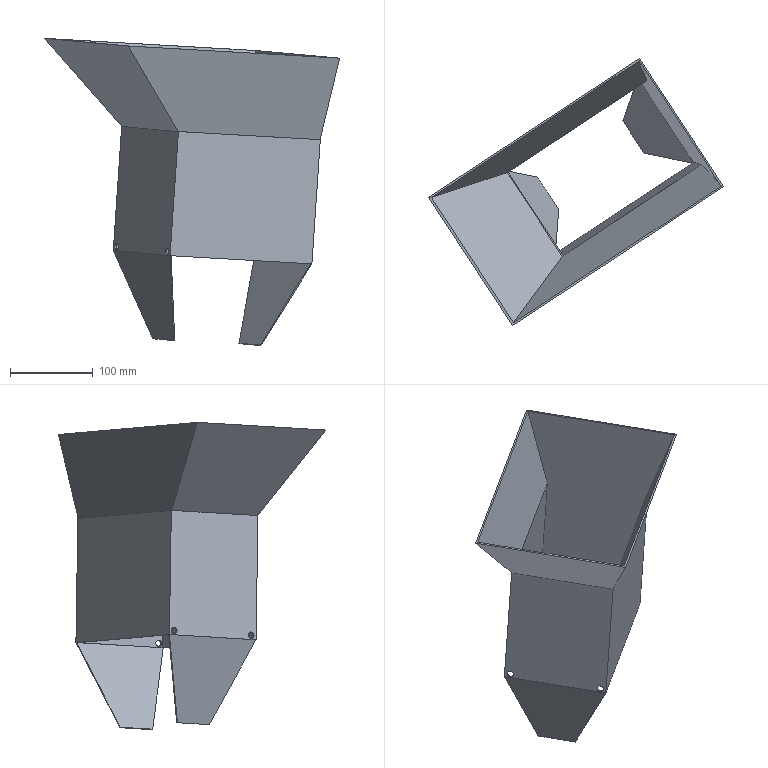Component | SolidWorks | MaterialChannel-1 | 1 solid | 37 faces | box 355.68 x 322.15 x 370.35 mm | volume 401352 mm3 | plane 29 | cylinder 8 | commonest cylinder face diameters 8 x8 | material AISI 304
STEP:
#1=COLOUR_RGB('',0.7922,0.8196,0.9333);
#2=FILL_AREA_STYLE_COLOUR('',#1);
#3=FILL_AREA_STYLE('',(#2));
#4=SURFACE_STYLE_FILL_AREA(#3);
#5=SURFACE_SIDE_STYLE('',(#4));
#6=SURFACE_STYLE_USAGE(.BOTH.,#5);
#7=PRESENTATION_STYLE_ASSIGNMENT((#6));
#8=CARTESIAN_POINT('',(-10.12,-1.207,26.784));
#9=VERTEX_POINT('',#8);
#10=CARTESIAN_POINT('',(-10.292,-0.9443,26.8));
#11=VERTEX_POINT('',#10);
#12=CARTESIAN_POINT('',(-10.206,-1.076,26.792));
#13=DIRECTION('',(0.8341,0.5496,-0.04788));
#14=DIRECTION('',(-0.5475,0.8353,0.05005));
#15=AXIS2_PLACEMENT_3D('',#12,#13,#14);
#16=CIRCLE('',#15,0.1575);
#17=EDGE_CURVE('',#9,#11,#16,.T.);
#18=ORIENTED_EDGE('',*,*,#17,.T.);
#19=CARTESIAN_POINT('',(-10.358,-0.9876,26.804));
#20=VERTEX_POINT('',#19);
#21=CARTESIAN_POINT('',(-3.626,3.448,26.418));
#22=DIRECTION('',(-0.8341,-0.5496,0.04788));
#23=VECTOR('',#22,39.37);
#24=LINE('',#21,#23);
#25=EDGE_CURVE('',#11,#20,#24,.T.);
#26=ORIENTED_EDGE('',*,*,#25,.T.);
#27=CARTESIAN_POINT('',(-10.186,-1.251,26.788));
#28=VERTEX_POINT('',#27);
#29=CARTESIAN_POINT('',(-10.272,-1.119,26.796));
#30=DIRECTION('',(-0.8341,-0.5496,0.04788));
#31=DIRECTION('',(0.5475,-0.8353,-0.05005));
#32=AXIS2_PLACEMENT_3D('',#29,#30,#31);
#33=CIRCLE('',#32,0.1575);
#34=EDGE_CURVE('',#20,#28,#33,.T.);
#35=ORIENTED_EDGE('',*,*,#34,.T.);
#36=CARTESIAN_POINT('',(-3.454,3.185,26.402));
#37=DIRECTION('',(-0.8341,-0.5496,0.04788));
#38=VECTOR('',#37,39.37);
#39=LINE('',#36,#38);
#40=EDGE_CURVE('',#9,#28,#39,.T.);
#41=ORIENTED_EDGE('',*,*,#40,.F.);
#42=EDGE_LOOP('',(#18,#26,#35,#41));
#43=FACE_OUTER_BOUND('',#42,.T.);
#44=CARTESIAN_POINT('',(-3.54,3.317,26.41));
#45=DIRECTION('',(-0.8341,-0.5496,0.04788));
#46=DIRECTION('',(0.5475,-0.8353,-0.05005));
#47=AXIS2_PLACEMENT_3D('',#44,#45,#46);
#48=CYLINDRICAL_SURFACE('',#47,0.1575);
#49=ADVANCED_FACE('',(#43),#48,.F.);
#50=CARTESIAN_POINT('',(-3.626,3.448,26.418));
#51=VERTEX_POINT('',#50);
#52=CARTESIAN_POINT('',(-3.454,3.185,26.402));
#53=VERTEX_POINT('',#52);
#54=CARTESIAN_POINT('',(-3.54,3.317,26.41));
#55=DIRECTION('',(-0.8341,-0.5496,0.04788));
#56=DIRECTION('',(0.5475,-0.8353,-0.05005));
#57=AXIS2_PLACEMENT_3D('',#54,#55,#56);
#58=CIRCLE('',#57,0.1575);
#59=EDGE_CURVE('',#51,#53,#58,.T.);
#60=ORIENTED_EDGE('',*,*,#59,.F.);
#61=CARTESIAN_POINT('',(-3.692,3.405,26.421));
#62=VERTEX_POINT('',#61);
#63=CARTESIAN_POINT('',(-3.626,3.448,26.418));
#64=DIRECTION('',(-0.8341,-0.5496,0.04788));
#65=VECTOR('',#64,39.37);
#66=LINE('',#63,#65);
#67=EDGE_CURVE('',#51,#62,#66,.T.);
#68=ORIENTED_EDGE('',*,*,#67,.T.);
#69=CARTESIAN_POINT('',(-3.52,3.142,26.406));
#70=VERTEX_POINT('',#69);
#71=CARTESIAN_POINT('',(-3.606,3.273,26.413));
#72=DIRECTION('',(-0.8341,-0.5496,0.04788));
#73=DIRECTION('',(0.5475,-0.8353,-0.05005));
#74=AXIS2_PLACEMENT_3D('',#71,#72,#73);
#75=CIRCLE('',#74,0.1575);
#76=EDGE_CURVE('',#62,#70,#75,.T.);
#77=ORIENTED_EDGE('',*,*,#76,.T.);
#78=CARTESIAN_POINT('',(-3.454,3.185,26.402));
#79=DIRECTION('',(-0.8341,-0.5496,0.04788));
#80=VECTOR('',#79,39.37);
#81=LINE('',#78,#80);
#82=EDGE_CURVE('',#53,#70,#81,.T.);
#83=ORIENTED_EDGE('',*,*,#82,.F.);
#84=EDGE_LOOP('',(#60,#68,#77,#83));
#85=FACE_OUTER_BOUND('',#84,.T.);
#86=CARTESIAN_POINT('',(-3.54,3.317,26.41));
#87=DIRECTION('',(-0.8341,-0.5496,0.04788));
#88=DIRECTION('',(0.5475,-0.8353,-0.05005));
#89=AXIS2_PLACEMENT_3D('',#86,#87,#88);
#90=CYLINDRICAL_SURFACE('',#89,0.1575);
#91=ADVANCED_FACE('',(#85),#90,.F.);
#92=CARTESIAN_POINT('',(-12.513,2.443,27.003));
#93=VERTEX_POINT('',#92);
#94=CARTESIAN_POINT('',(-12.685,2.706,27.019));
#95=VERTEX_POINT('',#94);
#96=CARTESIAN_POINT('',(-12.599,2.574,27.011));
#97=DIRECTION('',(0.8341,0.5496,-0.04788));
#98=DIRECTION('',(-0.5475,0.8353,0.05005));
#99=AXIS2_PLACEMENT_3D('',#96,#97,#98);
#100=CIRCLE('',#99,0.1575);
#101=EDGE_CURVE('',#93,#95,#100,.T.);
#102=ORIENTED_EDGE('',*,*,#101,.T.);
#103=CARTESIAN_POINT('',(-12.751,2.663,27.023));
#104=VERTEX_POINT('',#103);
#105=CARTESIAN_POINT('',(-6.019,7.098,26.636));
#106=DIRECTION('',(-0.8341,-0.5496,0.04788));
#107=VECTOR('',#106,39.37);
#108=LINE('',#105,#107);
#109=EDGE_CURVE('',#95,#104,#108,.T.);
#110=ORIENTED_EDGE('',*,*,#109,.T.);
#111=CARTESIAN_POINT('',(-12.578,2.4,27.007));
#112=VERTEX_POINT('',#111);
#113=CARTESIAN_POINT('',(-12.664,2.531,27.015));
#114=DIRECTION('',(-0.8341,-0.5496,0.04788));
#115=DIRECTION('',(0.5475,-0.8353,-0.05005));
#116=AXIS2_PLACEMENT_3D('',#113,#114,#115);
#117=CIRCLE('',#116,0.1575);
#118=EDGE_CURVE('',#104,#112,#117,.T.);
#119=ORIENTED_EDGE('',*,*,#118,.T.);
#120=CARTESIAN_POINT('',(-5.847,6.835,26.621));
#121=DIRECTION('',(-0.8341,-0.5496,0.04788));
#122=VECTOR('',#121,39.37);
#123=LINE('',#120,#122);
#124=EDGE_CURVE('',#93,#112,#123,.T.);
#125=ORIENTED_EDGE('',*,*,#124,.F.);
#126=EDGE_LOOP('',(#102,#110,#119,#125));
#127=FACE_OUTER_BOUND('',#126,.T.);
#128=CARTESIAN_POINT('',(-5.933,6.967,26.628));
#129=DIRECTION('',(-0.8341,-0.5496,0.04788));
#130=DIRECTION('',(0.5475,-0.8353,-0.05005));
#131=AXIS2_PLACEMENT_3D('',#128,#129,#130);
#132=CYLINDRICAL_SURFACE('',#131,0.1575);
#133=ADVANCED_FACE('',(#127),#132,.F.);
#134=CARTESIAN_POINT('',(-6.019,7.098,26.636));
#135=VERTEX_POINT('',#134);
#136=CARTESIAN_POINT('',(-5.847,6.835,26.621));
#137=VERTEX_POINT('',#136);
#138=CARTESIAN_POINT('',(-5.933,6.967,26.628));
#139=DIRECTION('',(-0.8341,-0.5496,0.04788));
#140=DIRECTION('',(0.5475,-0.8353,-0.05005));
#141=AXIS2_PLACEMENT_3D('',#138,#139,#140);
#142=CIRCLE('',#141,0.1575);
#143=EDGE_CURVE('',#135,#137,#142,.T.);
#144=ORIENTED_EDGE('',*,*,#143,.F.);
#145=CARTESIAN_POINT('',(-6.085,7.055,26.64));
#146=VERTEX_POINT('',#145);
#147=CARTESIAN_POINT('',(-6.019,7.098,26.636));
#148=DIRECTION('',(-0.8341,-0.5496,0.04788));
#149=VECTOR('',#148,39.37);
#150=LINE('',#147,#149);
#151=EDGE_CURVE('',#135,#146,#150,.T.);
#152=ORIENTED_EDGE('',*,*,#151,.T.);
#153=CARTESIAN_POINT('',(-5.912,6.792,26.624));
#154=VERTEX_POINT('',#153);
#155=CARTESIAN_POINT('',(-5.999,6.924,26.632));
#156=DIRECTION('',(-0.8341,-0.5496,0.04788));
#157=DIRECTION('',(0.5475,-0.8353,-0.05005));
#158=AXIS2_PLACEMENT_3D('',#155,#156,#157);
#159=CIRCLE('',#158,0.1575);
#160=EDGE_CURVE('',#146,#154,#159,.T.);
#161=ORIENTED_EDGE('',*,*,#160,.T.);
#162=CARTESIAN_POINT('',(-5.847,6.835,26.621));
#163=DIRECTION('',(-0.8341,-0.5496,0.04788));
#164=VECTOR('',#163,39.37);
#165=LINE('',#162,#164);
#166=EDGE_CURVE('',#137,#154,#165,.T.);
#167=ORIENTED_EDGE('',*,*,#166,.F.);
#168=EDGE_LOOP('',(#144,#152,#161,#167));
#169=FACE_OUTER_BOUND('',#168,.T.);
#170=CARTESIAN_POINT('',(-5.933,6.967,26.628));
#171=DIRECTION('',(-0.8341,-0.5496,0.04788));
#172=DIRECTION('',(0.5475,-0.8353,-0.05005));
#173=AXIS2_PLACEMENT_3D('',#170,#171,#172);
#174=CYLINDRICAL_SURFACE('',#173,0.1575);
#175=ADVANCED_FACE('',(#169),#174,.F.);
#176=CARTESIAN_POINT('',(-9.708,-1.33,32.556));
#177=VERTEX_POINT('',#176);
#178=CARTESIAN_POINT('',(-3.107,3.019,32.177));
#179=VERTEX_POINT('',#178);
#180=CARTESIAN_POINT('',(-3.107,3.019,32.177));
#181=DIRECTION('',(0.8341,0.5496,-0.04788));
#182=VECTOR('',#181,39.37);
#183=LINE('',#180,#182);
#184=EDGE_CURVE('',#177,#179,#183,.T.);
#185=ORIENTED_EDGE('',*,*,#184,.F.);
#186=CARTESIAN_POINT('',(-12.316,2.649,32.794));
#187=VERTEX_POINT('',#186);
#188=CARTESIAN_POINT('',(-9.708,-1.33,32.556));
#189=DIRECTION('',(0.5475,-0.8353,-0.05005));
#190=VECTOR('',#189,39.37);
#191=LINE('',#188,#190);
#192=EDGE_CURVE('',#187,#177,#191,.T.);
#193=ORIENTED_EDGE('',*,*,#192,.F.);
#194=CARTESIAN_POINT('',(-5.716,6.998,32.416));
#195=VERTEX_POINT('',#194);
#196=CARTESIAN_POINT('',(-12.316,2.649,32.794));
#197=DIRECTION('',(-0.8341,-0.5496,0.04788));
#198=VECTOR('',#197,39.37);
#199=LINE('',#196,#198);
#200=EDGE_CURVE('',#195,#187,#199,.T.);
#201=ORIENTED_EDGE('',*,*,#200,.F.);
#202=CARTESIAN_POINT('',(-5.716,6.999,32.416));
#203=VERTEX_POINT('',#202);
#204=CARTESIAN_POINT('',(-5.759,7.064,32.419));
#205=DIRECTION('',(0.5475,-0.8353,-0.05005));
#206=VECTOR('',#205,39.37);
#207=LINE('',#204,#206);
#208=EDGE_CURVE('',#203,#195,#207,.T.);
#209=ORIENTED_EDGE('',*,*,#208,.F.);
#210=CARTESIAN_POINT('',(-12.355,2.624,32.797));
#211=VERTEX_POINT('',#210);
#212=CARTESIAN_POINT('',(-15.666,0.4426,32.987));
#213=DIRECTION('',(0.8341,0.5496,-0.04788));
#214=VECTOR('',#213,39.37);
#215=LINE('',#212,#214);
#216=EDGE_CURVE('',#211,#203,#215,.T.);
#217=ORIENTED_EDGE('',*,*,#216,.F.);
#218=CARTESIAN_POINT('',(-9.746,-1.356,32.558));
#219=VERTEX_POINT('',#218);
#220=CARTESIAN_POINT('',(-9.714,-1.405,32.555));
#221=DIRECTION('',(0.5475,-0.8353,-0.05005));
#222=VECTOR('',#221,39.37);
#223=LINE('',#220,#222);
#224=EDGE_CURVE('',#211,#219,#223,.T.);
#225=ORIENTED_EDGE('',*,*,#224,.T.);
#226=CARTESIAN_POINT('',(-3.107,3.018,32.177));
#227=VERTEX_POINT('',#226);
#228=CARTESIAN_POINT('',(-13.057,-3.538,32.748));
#229=DIRECTION('',(-0.8341,-0.5496,0.04788));
#230=VECTOR('',#229,39.37);
#231=LINE('',#228,#230);
#232=EDGE_CURVE('',#227,#219,#231,.T.);
#233=ORIENTED_EDGE('',*,*,#232,.F.);
#234=CARTESIAN_POINT('',(-5.759,7.064,32.419));
#235=DIRECTION('',(0.5475,-0.8353,-0.05005));
#236=VECTOR('',#235,39.37);
#237=LINE('',#234,#236);
#238=EDGE_CURVE('',#179,#227,#237,.T.);
#239=ORIENTED_EDGE('',*,*,#238,.F.);
#240=EDGE_LOOP('',(#185,#193,#201,#209,#217,#225,#233,#239));
#241=FACE_OUTER_BOUND('',#240,.T.);
#242=CARTESIAN_POINT('',(-13.025,-3.586,32.745));
#243=DIRECTION('',(-0.0675,0.01553,-0.9976));
#244=DIRECTION('',(-0.8341,-0.5496,0.04788));
#245=AXIS2_PLACEMENT_3D('',#242,#243,#244);
#246=PLANE('',#245);
#247=ADVANCED_FACE('',(#241),#246,.F.);
#248=CARTESIAN_POINT('',(-6.079,8.034,36.324));
#249=VERTEX_POINT('',#248);
#250=CARTESIAN_POINT('',(-2.091,1.95,35.959));
#251=VERTEX_POINT('',#250);
#252=CARTESIAN_POINT('',(-2.091,1.95,35.959));
#253=DIRECTION('',(0.5475,-0.8353,-0.05005));
#254=VECTOR('',#253,39.37);
#255=LINE('',#252,#254);
#256=EDGE_CURVE('',#249,#251,#255,.T.);
#257=ORIENTED_EDGE('',*,*,#256,.F.);
#258=CARTESIAN_POINT('',(-16.095,1.434,36.899));
#259=VERTEX_POINT('',#258);
#260=CARTESIAN_POINT('',(-16.095,1.434,36.899));
#261=DIRECTION('',(0.8341,0.5496,-0.04788));
#262=VECTOR('',#261,39.37);
#263=LINE('',#260,#262);
#264=EDGE_CURVE('',#259,#249,#263,.T.);
#265=ORIENTED_EDGE('',*,*,#264,.F.);
#266=CARTESIAN_POINT('',(-12.107,-4.649,36.534));
#267=VERTEX_POINT('',#266);
#268=CARTESIAN_POINT('',(-12.107,-4.649,36.534));
#269=DIRECTION('',(0.5475,-0.8353,-0.05005));
#270=VECTOR('',#269,39.37);
#271=LINE('',#268,#270);
#272=EDGE_CURVE('',#259,#267,#271,.T.);
#273=ORIENTED_EDGE('',*,*,#272,.T.);
#274=CARTESIAN_POINT('',(-12.107,-4.649,36.534));
#275=DIRECTION('',(0.8341,0.5496,-0.04788));
#276=VECTOR('',#275,39.37);
#277=LINE('',#274,#276);
#278=EDGE_CURVE('',#267,#251,#277,.T.);
#279=ORIENTED_EDGE('',*,*,#278,.T.);
#280=EDGE_LOOP('',(#257,#265,#273,#279));
#281=FACE_OUTER_BOUND('',#280,.T.);
#282=CARTESIAN_POINT('',(-15.957,1.427,36.889));
#283=VERTEX_POINT('',#282);
#284=CARTESIAN_POINT('',(-6.1,7.922,36.323));
#285=VERTEX_POINT('',#284);
#286=CARTESIAN_POINT('',(-16.05,1.366,36.895));
#287=DIRECTION('',(0.8341,0.5496,-0.04788));
#288=VECTOR('',#287,39.37);
#289=LINE('',#286,#288);
#290=EDGE_CURVE('',#283,#285,#289,.T.);
#291=ORIENTED_EDGE('',*,*,#290,.T.);
#292=CARTESIAN_POINT('',(-2.202,1.975,35.967));
#293=VERTEX_POINT('',#292);
#294=CARTESIAN_POINT('',(-2.157,1.907,35.963));
#295=DIRECTION('',(0.5475,-0.8353,-0.05005));
#296=VECTOR('',#295,39.37);
#297=LINE('',#294,#296);
#298=EDGE_CURVE('',#285,#293,#297,.T.);
#299=ORIENTED_EDGE('',*,*,#298,.T.);
#300=CARTESIAN_POINT('',(-12.059,-4.519,36.533));
#301=VERTEX_POINT('',#300);
#302=CARTESIAN_POINT('',(-12.152,-4.581,36.538));
#303=DIRECTION('',(0.8341,0.5496,-0.04788));
#304=VECTOR('',#303,39.37);
#305=LINE('',#302,#304);
#306=EDGE_CURVE('',#301,#293,#305,.T.);
#307=ORIENTED_EDGE('',*,*,#306,.F.);
#308=CARTESIAN_POINT('',(-11.691,-5.081,36.499));
#309=DIRECTION('',(0.5475,-0.8353,-0.05005));
#310=VECTOR('',#309,39.37);
#311=LINE('',#308,#310);
#312=EDGE_CURVE('',#283,#301,#311,.T.);
#313=ORIENTED_EDGE('',*,*,#312,.F.);
#314=EDGE_LOOP('',(#291,#299,#307,#313));
#315=FACE_BOUND('',#314,.T.);
#316=CARTESIAN_POINT('',(-12.107,-4.649,36.534));
#317=DIRECTION('',(0.0675,-0.01553,0.9976));
#318=DIRECTION('',(0.8341,0.5496,-0.04788));
#319=AXIS2_PLACEMENT_3D('',#316,#317,#318);
#320=PLANE('',#319);
#321=ADVANCED_FACE('',(#281,#315),#320,.T.);
#322=CARTESIAN_POINT('',(-12.43,2.673,32.724));
#323=VERTEX_POINT('',#322);
#324=CARTESIAN_POINT('',(-12.419,2.656,32.723));
#325=VERTEX_POINT('',#324);
#326=CARTESIAN_POINT('',(-12.43,2.673,32.724));
#327=DIRECTION('',(0.5475,-0.8353,-0.05005));
#328=VECTOR('',#327,39.37);
#329=LINE('',#326,#328);
#330=EDGE_CURVE('',#323,#325,#329,.T.);
#331=ORIENTED_EDGE('',*,*,#330,.T.);
#332=CARTESIAN_POINT('',(-5.688,7.092,32.336));
#333=VERTEX_POINT('',#332);
#334=CARTESIAN_POINT('',(-15.703,0.4926,32.911));
#335=DIRECTION('',(0.8341,0.5496,-0.04788));
#336=VECTOR('',#335,39.37);
#337=LINE('',#334,#336);
#338=EDGE_CURVE('',#325,#333,#337,.T.);
#339=ORIENTED_EDGE('',*,*,#338,.T.);
#340=CARTESIAN_POINT('',(-5.698,7.108,32.337));
#341=VERTEX_POINT('',#340);
#342=CARTESIAN_POINT('',(-5.698,7.108,32.337));
#343=DIRECTION('',(-0.5475,0.8353,0.05005));
#344=VECTOR('',#343,39.37);
#345=LINE('',#342,#344);
#346=EDGE_CURVE('',#333,#341,#345,.T.);
#347=ORIENTED_EDGE('',*,*,#346,.T.);
#348=CARTESIAN_POINT('',(-12.43,2.673,32.724));
#349=DIRECTION('',(-0.8341,-0.5496,0.04788));
#350=VECTOR('',#349,39.37);
#351=LINE('',#348,#350);
#352=EDGE_CURVE('',#341,#323,#351,.T.);
#353=ORIENTED_EDGE('',*,*,#352,.T.);
#354=EDGE_LOOP('',(#331,#339,#347,#353));
#355=FACE_OUTER_BOUND('',#354,.T.);
#356=CARTESIAN_POINT('',(-12.43,2.673,32.724));
#357=DIRECTION('',(0.0675,-0.01553,0.9976));
#358=DIRECTION('',(0.8341,0.5496,-0.04788));
#359=AXIS2_PLACEMENT_3D('',#356,#357,#358);
#360=PLANE('',#359);
#361=ADVANCED_FACE('',(#355),#360,.T.);
#362=CARTESIAN_POINT('',(-6.12,7.091,26.446));
#363=VERTEX_POINT('',#362);
#364=CARTESIAN_POINT('',(-12.72,2.742,26.825));
#365=VERTEX_POINT('',#364);
#366=CARTESIAN_POINT('',(-12.72,2.742,26.825));
#367=DIRECTION('',(-0.8341,-0.5496,0.04788));
#368=VECTOR('',#367,39.37);
#369=LINE('',#366,#368);
#370=EDGE_CURVE('',#363,#365,#369,.T.);
#371=ORIENTED_EDGE('',*,*,#370,.T.);
#372=CARTESIAN_POINT('',(-10.112,-1.237,26.586));
#373=VERTEX_POINT('',#372);
#374=CARTESIAN_POINT('',(-12.72,2.742,26.825));
#375=DIRECTION('',(0.5475,-0.8353,-0.05005));
#376=VECTOR('',#375,39.37);
#377=LINE('',#374,#376);
#378=EDGE_CURVE('',#365,#373,#377,.T.);
#379=ORIENTED_EDGE('',*,*,#378,.T.);
#380=CARTESIAN_POINT('',(-3.511,3.112,26.207));
#381=VERTEX_POINT('',#380);
#382=CARTESIAN_POINT('',(-10.112,-1.237,26.586));
#383=DIRECTION('',(0.8341,0.5496,-0.04788));
#384=VECTOR('',#383,39.37);
#385=LINE('',#382,#384);
#386=EDGE_CURVE('',#373,#381,#385,.T.);
#387=ORIENTED_EDGE('',*,*,#386,.T.);
#388=CARTESIAN_POINT('',(-6.12,7.091,26.446));
#389=DIRECTION('',(-0.5475,0.8353,0.05005));
#390=VECTOR('',#389,39.37);
#391=LINE('',#388,#390);
#392=EDGE_CURVE('',#381,#363,#391,.T.);
#393=ORIENTED_EDGE('',*,*,#392,.T.);
#394=EDGE_LOOP('',(#371,#379,#387,#393));
#395=FACE_BOUND('',#394,.T.);
#396=CARTESIAN_POINT('',(-6.146,7.168,26.449));
#397=VERTEX_POINT('',#396);
#398=CARTESIAN_POINT('',(-12.779,2.797,26.829));
#399=VERTEX_POINT('',#398);
#400=CARTESIAN_POINT('',(-12.829,2.764,26.832));
#401=DIRECTION('',(-0.8341,-0.5496,0.04788));
#402=VECTOR('',#401,39.37);
#403=LINE('',#400,#402);
#404=EDGE_CURVE('',#397,#399,#403,.T.);
#405=ORIENTED_EDGE('',*,*,#404,.F.);
#406=CARTESIAN_POINT('',(-3.452,3.057,26.202));
#407=VERTEX_POINT('',#406);
#408=CARTESIAN_POINT('',(-8.528,10.802,26.666));
#409=DIRECTION('',(0.5475,-0.8353,-0.05005));
#410=VECTOR('',#409,39.37);
#411=LINE('',#408,#410);
#412=EDGE_CURVE('',#397,#407,#411,.T.);
#413=ORIENTED_EDGE('',*,*,#412,.T.);
#414=CARTESIAN_POINT('',(-10.085,-1.314,26.583));
#415=VERTEX_POINT('',#414);
#416=CARTESIAN_POINT('',(-10.134,-1.346,26.586));
#417=DIRECTION('',(0.8341,0.5496,-0.04788));
#418=VECTOR('',#417,39.37);
#419=LINE('',#416,#418);
#420=EDGE_CURVE('',#415,#407,#419,.T.);
#421=ORIENTED_EDGE('',*,*,#420,.F.);
#422=CARTESIAN_POINT('',(-15.162,6.431,27.047));
#423=DIRECTION('',(0.5475,-0.8353,-0.05005));
#424=VECTOR('',#423,39.37);
#425=LINE('',#422,#424);
#426=EDGE_CURVE('',#399,#415,#425,.T.);
#427=ORIENTED_EDGE('',*,*,#426,.F.);
#428=EDGE_LOOP('',(#405,#413,#421,#427));
#429=FACE_OUTER_BOUND('',#428,.T.);
#430=CARTESIAN_POINT('',(-12.829,2.764,26.832));
#431=DIRECTION('',(0.0675,-0.01553,0.9976));
#432=DIRECTION('',(0.8341,0.5496,-0.04788));
#433=AXIS2_PLACEMENT_3D('',#430,#431,#432);
#434=PLANE('',#433);
#435=ADVANCED_FACE('',(#395,#429),#434,.F.);
#436=CARTESIAN_POINT('',(-9.746,-1.422,32.478));
#437=VERTEX_POINT('',#436);
#438=CARTESIAN_POINT('',(-3.015,3.014,32.092));
#439=VERTEX_POINT('',#438);
#440=CARTESIAN_POINT('',(-13.03,-3.585,32.667));
#441=DIRECTION('',(0.8341,0.5496,-0.04788));
#442=VECTOR('',#441,39.37);
#443=LINE('',#440,#442);
#444=EDGE_CURVE('',#437,#439,#443,.T.);
#445=ORIENTED_EDGE('',*,*,#444,.F.);
#446=CARTESIAN_POINT('',(-9.736,-1.438,32.477));
#447=VERTEX_POINT('',#446);
#448=CARTESIAN_POINT('',(-12.43,2.673,32.724));
#449=DIRECTION('',(0.5475,-0.8353,-0.05005));
#450=VECTOR('',#449,39.37);
#451=LINE('',#448,#450);
#452=EDGE_CURVE('',#437,#447,#451,.T.);
#453=ORIENTED_EDGE('',*,*,#452,.T.);
#454=CARTESIAN_POINT('',(-3.004,2.998,32.091));
#455=VERTEX_POINT('',#454);
#456=CARTESIAN_POINT('',(-9.736,-1.438,32.477));
#457=DIRECTION('',(0.8341,0.5496,-0.04788));
#458=VECTOR('',#457,39.37);
#459=LINE('',#456,#458);
#460=EDGE_CURVE('',#447,#455,#459,.T.);
#461=ORIENTED_EDGE('',*,*,#460,.T.);
#462=CARTESIAN_POINT('',(-5.698,7.108,32.337));
#463=DIRECTION('',(-0.5475,0.8353,0.05005));
#464=VECTOR('',#463,39.37);
#465=LINE('',#462,#464);
#466=EDGE_CURVE('',#455,#439,#465,.T.);
#467=ORIENTED_EDGE('',*,*,#466,.T.);
#468=EDGE_LOOP('',(#445,#453,#461,#467));
#469=FACE_OUTER_BOUND('',#468,.T.);
#470=CARTESIAN_POINT('',(-12.43,2.673,32.724));
#471=DIRECTION('',(0.0675,-0.01553,0.9976));
#472=DIRECTION('',(0.8341,0.5496,-0.04788));
#473=AXIS2_PLACEMENT_3D('',#470,#471,#472);
#474=PLANE('',#473);
#475=ADVANCED_FACE('',(#469),#474,.T.);
#476=CARTESIAN_POINT('',(-10.272,-1.119,26.796));
#477=DIRECTION('',(-0.8341,-0.5496,0.04788));
#478=DIRECTION('',(0.5475,-0.8353,-0.05005));
#479=AXIS2_PLACEMENT_3D('',#476,#477,#478);
#480=CIRCLE('',#479,0.1575);
#481=EDGE_CURVE('',#28,#20,#480,.T.);
#482=ORIENTED_EDGE('',*,*,#481,.F.);
#483=ORIENTED_EDGE('',*,*,#34,.F.);
#484=EDGE_LOOP('',(#482,#483));
#485=FACE_BOUND('',#484,.T.);
#486=CARTESIAN_POINT('',(-12.664,2.531,27.015));
#487=DIRECTION('',(-0.8341,-0.5496,0.04788));
#488=DIRECTION('',(0.5475,-0.8353,-0.05005));
#489=AXIS2_PLACEMENT_3D('',#486,#487,#488);
#490=CIRCLE('',#489,0.1575);
#491=EDGE_CURVE('',#112,#104,#490,.T.);
#492=ORIENTED_EDGE('',*,*,#491,.F.);
#493=ORIENTED_EDGE('',*,*,#118,.F.);
#494=EDGE_LOOP('',(#492,#493));
#495=FACE_BOUND('',#494,.T.);
#496=CARTESIAN_POINT('',(-12.829,2.764,26.832));
#497=VERTEX_POINT('',#496);
#498=CARTESIAN_POINT('',(-10.134,-1.346,26.586));
#499=VERTEX_POINT('',#498);
#500=CARTESIAN_POINT('',(-12.829,2.764,26.832));
#501=DIRECTION('',(0.5475,-0.8353,-0.05005));
#502=VECTOR('',#501,39.37);
#503=LINE('',#500,#502);
#504=EDGE_CURVE('',#497,#499,#503,.T.);
#505=ORIENTED_EDGE('',*,*,#504,.T.);
#506=CARTESIAN_POINT('',(-9.736,-1.438,32.477));
#507=DIRECTION('',(-0.0675,0.01553,-0.9976));
#508=VECTOR('',#507,39.37);
#509=LINE('',#506,#508);
#510=EDGE_CURVE('',#447,#499,#509,.T.);
#511=ORIENTED_EDGE('',*,*,#510,.F.);
#512=ORIENTED_EDGE('',*,*,#452,.F.);
#513=CARTESIAN_POINT('',(-12.43,2.673,32.724));
#514=DIRECTION('',(0.5475,-0.8353,-0.05005));
#515=VECTOR('',#514,39.37);
#516=LINE('',#513,#515);
#517=EDGE_CURVE('',#325,#437,#516,.T.);
#518=ORIENTED_EDGE('',*,*,#517,.F.);
#519=ORIENTED_EDGE('',*,*,#330,.F.);
#520=CARTESIAN_POINT('',(-12.43,2.673,32.724));
#521=DIRECTION('',(-0.0675,0.01553,-0.9976));
#522=VECTOR('',#521,39.37);
#523=LINE('',#520,#522);
#524=EDGE_CURVE('',#323,#497,#523,.T.);
#525=ORIENTED_EDGE('',*,*,#524,.T.);
#526=EDGE_LOOP('',(#505,#511,#512,#518,#519,#525));
#527=FACE_OUTER_BOUND('',#526,.T.);
#528=CARTESIAN_POINT('',(-12.43,2.673,32.724));
#529=DIRECTION('',(0.8341,0.5496,-0.04788));
#530=DIRECTION('',(-0.5475,0.8353,0.05005));
#531=AXIS2_PLACEMENT_3D('',#528,#529,#530);
#532=PLANE('',#531);
#533=ADVANCED_FACE('',(#485,#495,#527),#532,.F.);
#534=ORIENTED_EDGE('',*,*,#510,.T.);
#535=CARTESIAN_POINT('',(-3.403,3.089,26.2));
#536=DIRECTION('',(-0.8341,-0.5496,0.04788));
#537=VECTOR('',#536,39.37);
#538=LINE('',#535,#537);
#539=EDGE_CURVE('',#415,#499,#538,.T.);
#540=ORIENTED_EDGE('',*,*,#539,.F.);
#541=ORIENTED_EDGE('',*,*,#420,.T.);
#542=CARTESIAN_POINT('',(-3.403,3.089,26.2));
#543=VERTEX_POINT('',#542);
#544=CARTESIAN_POINT('',(-3.403,3.089,26.2));
#545=DIRECTION('',(-0.8341,-0.5496,0.04788));
#546=VECTOR('',#545,39.37);
#547=LINE('',#544,#546);
#548=EDGE_CURVE('',#543,#407,#547,.T.);
#549=ORIENTED_EDGE('',*,*,#548,.F.);
#550=CARTESIAN_POINT('',(-3.004,2.998,32.091));
#551=DIRECTION('',(-0.0675,0.01553,-0.9976));
#552=VECTOR('',#551,39.37);
#553=LINE('',#550,#552);
#554=EDGE_CURVE('',#455,#543,#553,.T.);
#555=ORIENTED_EDGE('',*,*,#554,.F.);
#556=ORIENTED_EDGE('',*,*,#460,.F.);
#557=EDGE_LOOP('',(#534,#540,#541,#549,#555,#556));
#558=FACE_OUTER_BOUND('',#557,.T.);
#559=CARTESIAN_POINT('',(-9.736,-1.438,32.477));
#560=DIRECTION('',(-0.5475,0.8353,0.05005));
#561=DIRECTION('',(0.0675,-0.01553,0.9976));
#562=AXIS2_PLACEMENT_3D('',#559,#560,#561);
#563=PLANE('',#562);
#564=ADVANCED_FACE('',(#558),#563,.F.);
#565=CARTESIAN_POINT('',(-3.54,3.317,26.41));
#566=DIRECTION('',(-0.8341,-0.5496,0.04788));
#567=DIRECTION('',(0.5475,-0.8353,-0.05005));
#568=AXIS2_PLACEMENT_3D('',#565,#566,#567);
#569=CIRCLE('',#568,0.1575);
#570=EDGE_CURVE('',#53,#51,#569,.T.);
#571=ORIENTED_EDGE('',*,*,#570,.T.);
#572=ORIENTED_EDGE('',*,*,#59,.T.);
#573=EDGE_LOOP('',(#571,#572));
#574=FACE_BOUND('',#573,.T.);
#575=CARTESIAN_POINT('',(-5.933,6.967,26.628));
#576=DIRECTION('',(-0.8341,-0.5496,0.04788));
#577=DIRECTION('',(0.5475,-0.8353,-0.05005));
#578=AXIS2_PLACEMENT_3D('',#575,#576,#577);
#579=CIRCLE('',#578,0.1575);
#580=EDGE_CURVE('',#137,#135,#579,.T.);
#581=ORIENTED_EDGE('',*,*,#580,.T.);
#582=ORIENTED_EDGE('',*,*,#143,.T.);
#583=EDGE_LOOP('',(#581,#582));
#584=FACE_BOUND('',#583,.T.);
#585=CARTESIAN_POINT('',(-6.097,7.2,26.446));
#586=VERTEX_POINT('',#585);
#587=CARTESIAN_POINT('',(-6.097,7.2,26.446));
#588=DIRECTION('',(-0.5475,0.8353,0.05005));
#589=VECTOR('',#588,39.37);
#590=LINE('',#587,#589);
#591=EDGE_CURVE('',#543,#586,#590,.T.);
#592=ORIENTED_EDGE('',*,*,#591,.T.);
#593=CARTESIAN_POINT('',(-5.698,7.108,32.337));
#594=DIRECTION('',(-0.0675,0.01553,-0.9976));
#595=VECTOR('',#594,39.37);
#596=LINE('',#593,#595);
#597=EDGE_CURVE('',#341,#586,#596,.T.);
#598=ORIENTED_EDGE('',*,*,#597,.F.);
#599=ORIENTED_EDGE('',*,*,#346,.F.);
#600=CARTESIAN_POINT('',(-6.079,8.034,36.324));
#601=DIRECTION('',(-0.09517,0.2288,0.9688));
#602=VECTOR('',#601,39.37);
#603=LINE('',#600,#602);
#604=EDGE_CURVE('',#333,#249,#603,.T.);
#605=ORIENTED_EDGE('',*,*,#604,.T.);
#606=ORIENTED_EDGE('',*,*,#256,.T.);
#607=CARTESIAN_POINT('',(-3.015,3.014,32.092));
#608=DIRECTION('',(-0.2243,0.2585,-0.9396));
#609=VECTOR('',#608,39.37);
#610=LINE('',#607,#609);
#611=EDGE_CURVE('',#251,#439,#610,.T.);
#612=ORIENTED_EDGE('',*,*,#611,.T.);
#613=ORIENTED_EDGE('',*,*,#466,.F.);
#614=ORIENTED_EDGE('',*,*,#554,.T.);
#615=EDGE_LOOP('',(#592,#598,#599,#605,#606,#612,#613,#614));
#616=FACE_OUTER_BOUND('',#615,.T.);
#617=CARTESIAN_POINT('',(-5.698,7.108,32.337));
#618=DIRECTION('',(-0.8341,-0.5496,0.04788));
#619=DIRECTION('',(0.5475,-0.8353,-0.05005));
#620=AXIS2_PLACEMENT_3D('',#617,#618,#619);
#621=PLANE('',#620);
#622=ADVANCED_FACE('',(#574,#584,#616),#621,.F.);
#623=ORIENTED_EDGE('',*,*,#597,.T.);
#624=CARTESIAN_POINT('',(-6.097,7.2,26.446));
#625=DIRECTION('',(-0.8341,-0.5496,0.04788));
#626=VECTOR('',#625,39.37);
#627=LINE('',#624,#626);
#628=EDGE_CURVE('',#586,#397,#627,.T.);
#629=ORIENTED_EDGE('',*,*,#628,.T.);
#630=ORIENTED_EDGE('',*,*,#404,.T.);
#631=CARTESIAN_POINT('',(-6.097,7.2,26.446));
#632=DIRECTION('',(-0.8341,-0.5496,0.04788));
#633=VECTOR('',#632,39.37);
#634=LINE('',#631,#633);
#635=EDGE_CURVE('',#399,#497,#634,.T.);
#636=ORIENTED_EDGE('',*,*,#635,.T.);
#637=ORIENTED_EDGE('',*,*,#524,.F.);
#638=ORIENTED_EDGE('',*,*,#352,.F.);
#639=EDGE_LOOP('',(#623,#629,#630,#636,#637,#638));
#640=FACE_OUTER_BOUND('',#639,.T.);
#641=CARTESIAN_POINT('',(-12.43,2.673,32.724));
#642=DIRECTION('',(0.5475,-0.8353,-0.05005));
#643=DIRECTION('',(-0.0675,0.01553,-0.9976));
#644=AXIS2_PLACEMENT_3D('',#641,#642,#643);
#645=PLANE('',#644);
#646=ADVANCED_FACE('',(#640),#645,.F.);
#647=ORIENTED_EDGE('',*,*,#370,.F.);
#648=CARTESIAN_POINT('',(-5.721,6.999,32.337));
#649=DIRECTION('',(-0.0675,0.01553,-0.9976));
#650=VECTOR('',#649,39.37);
#651=LINE('',#648,#650);
#652=EDGE_CURVE('',#195,#363,#651,.T.);
#653=ORIENTED_EDGE('',*,*,#652,.F.);
#654=ORIENTED_EDGE('',*,*,#200,.T.);
#655=CARTESIAN_POINT('',(-12.321,2.65,32.716));
#656=DIRECTION('',(-0.0675,0.01553,-0.9976));
#657=VECTOR('',#656,39.37);
#658=LINE('',#655,#657);
#659=EDGE_CURVE('',#187,#365,#658,.T.);
#660=ORIENTED_EDGE('',*,*,#659,.T.);
#661=EDGE_LOOP('',(#647,#653,#654,#660));
#662=FACE_OUTER_BOUND('',#661,.T.);
#663=CARTESIAN_POINT('',(-12.321,2.65,32.716));
#664=DIRECTION('',(0.5475,-0.8353,-0.05005));
#665=DIRECTION('',(-0.0675,0.01553,-0.9976));
#666=AXIS2_PLACEMENT_3D('',#663,#664,#665);
#667=PLANE('',#666);
#668=ADVANCED_FACE('',(#662),#667,.T.);
#669=ORIENTED_EDGE('',*,*,#17,.F.);
#670=CARTESIAN_POINT('',(-10.206,-1.076,26.792));
#671=DIRECTION('',(0.8341,0.5496,-0.04788));
#672=DIRECTION('',(-0.5475,0.8353,0.05005));
#673=AXIS2_PLACEMENT_3D('',#670,#671,#672);
#674=CIRCLE('',#673,0.1575);
#675=EDGE_CURVE('',#11,#9,#674,.T.);
#676=ORIENTED_EDGE('',*,*,#675,.F.);
#677=EDGE_LOOP('',(#669,#676));
#678=FACE_BOUND('',#677,.T.);
#679=ORIENTED_EDGE('',*,*,#101,.F.);
#680=CARTESIAN_POINT('',(-12.599,2.574,27.011));
#681=DIRECTION('',(0.8341,0.5496,-0.04788));
#682=DIRECTION('',(-0.5475,0.8353,0.05005));
#683=AXIS2_PLACEMENT_3D('',#680,#681,#682);
#684=CIRCLE('',#683,0.1575);
#685=EDGE_CURVE('',#95,#93,#684,.T.);
#686=ORIENTED_EDGE('',*,*,#685,.F.);
#687=EDGE_LOOP('',(#679,#686));
#688=FACE_BOUND('',#687,.T.);
#689=ORIENTED_EDGE('',*,*,#378,.F.);
#690=ORIENTED_EDGE('',*,*,#659,.F.);
#691=ORIENTED_EDGE('',*,*,#192,.T.);
#692=CARTESIAN_POINT('',(-9.713,-1.329,32.477));
#693=DIRECTION('',(-0.0675,0.01553,-0.9976));
#694=VECTOR('',#693,39.37);
#695=LINE('',#692,#694);
#696=EDGE_CURVE('',#177,#373,#695,.T.);
#697=ORIENTED_EDGE('',*,*,#696,.T.);
#698=EDGE_LOOP('',(#689,#690,#691,#697));
#699=FACE_OUTER_BOUND('',#698,.T.);
#700=CARTESIAN_POINT('',(-12.321,2.65,32.716));
#701=DIRECTION('',(0.8341,0.5496,-0.04788));
#702=DIRECTION('',(-0.5475,0.8353,0.05005));
#703=AXIS2_PLACEMENT_3D('',#700,#701,#702);
#704=PLANE('',#703);
#705=ADVANCED_FACE('',(#678,#688,#699),#704,.T.);
#706=ORIENTED_EDGE('',*,*,#386,.F.);
#707=ORIENTED_EDGE('',*,*,#696,.F.);
#708=ORIENTED_EDGE('',*,*,#184,.T.);
#709=CARTESIAN_POINT('',(-3.113,3.02,32.099));
#710=DIRECTION('',(-0.0675,0.01553,-0.9976));
#711=VECTOR('',#710,39.37);
#712=LINE('',#709,#711);
#713=EDGE_CURVE('',#179,#381,#712,.T.);
#714=ORIENTED_EDGE('',*,*,#713,.T.);
#715=EDGE_LOOP('',(#706,#707,#708,#714));
#716=FACE_OUTER_BOUND('',#715,.T.);
#717=CARTESIAN_POINT('',(-9.713,-1.329,32.477));
#718=DIRECTION('',(-0.5475,0.8353,0.05005));
#719=DIRECTION('',(0.0675,-0.01553,0.9976));
#720=AXIS2_PLACEMENT_3D('',#717,#718,#719);
#721=PLANE('',#720);
#722=ADVANCED_FACE('',(#716),#721,.T.);
#723=CARTESIAN_POINT('',(-3.606,3.273,26.413));
#724=DIRECTION('',(-0.8341,-0.5496,0.04788));
#725=DIRECTION('',(0.5475,-0.8353,-0.05005));
#726=AXIS2_PLACEMENT_3D('',#723,#724,#725);
#727=CIRCLE('',#726,0.1575);
#728=EDGE_CURVE('',#70,#62,#727,.T.);
#729=ORIENTED_EDGE('',*,*,#728,.F.);
#730=ORIENTED_EDGE('',*,*,#76,.F.);
#731=EDGE_LOOP('',(#729,#730));
#732=FACE_BOUND('',#731,.T.);
#733=CARTESIAN_POINT('',(-5.999,6.924,26.632));
#734=DIRECTION('',(-0.8341,-0.5496,0.04788));
#735=DIRECTION('',(0.5475,-0.8353,-0.05005));
#736=AXIS2_PLACEMENT_3D('',#733,#734,#735);
#737=CIRCLE('',#736,0.1575);
#738=EDGE_CURVE('',#154,#146,#737,.T.);
#739=ORIENTED_EDGE('',*,*,#738,.F.);
#740=ORIENTED_EDGE('',*,*,#160,.F.);
#741=EDGE_LOOP('',(#739,#740));
#742=FACE_BOUND('',#741,.T.);
#743=ORIENTED_EDGE('',*,*,#392,.F.);
#744=ORIENTED_EDGE('',*,*,#713,.F.);
#745=ORIENTED_EDGE('',*,*,#238,.T.);
#746=CARTESIAN_POINT('',(-3.12,3.033,32.122));
#747=DIRECTION('',(-0.2243,0.2585,-0.9396));
#748=VECTOR('',#747,39.37);
#749=LINE('',#746,#748);
#750=EDGE_CURVE('',#293,#227,#749,.T.);
#751=ORIENTED_EDGE('',*,*,#750,.F.);
#752=ORIENTED_EDGE('',*,*,#298,.F.);
#753=CARTESIAN_POINT('',(-6.102,7.927,36.347));
#754=DIRECTION('',(-0.09517,0.2288,0.9688));
#755=VECTOR('',#754,39.37);
#756=LINE('',#753,#755);
#757=EDGE_CURVE('',#203,#285,#756,.T.);
#758=ORIENTED_EDGE('',*,*,#757,.F.);
#759=ORIENTED_EDGE('',*,*,#208,.T.);
#760=ORIENTED_EDGE('',*,*,#652,.T.);
#761=EDGE_LOOP('',(#743,#744,#745,#751,#752,#758,#759,#760));
#762=FACE_OUTER_BOUND('',#761,.T.);
#763=CARTESIAN_POINT('',(-5.721,6.999,32.337));
#764=DIRECTION('',(-0.8341,-0.5496,0.04788));
#765=DIRECTION('',(0.5475,-0.8353,-0.05005));
#766=AXIS2_PLACEMENT_3D('',#763,#764,#765);
#767=PLANE('',#766);
#768=ADVANCED_FACE('',(#732,#742,#762),#767,.T.);
#769=ORIENTED_EDGE('',*,*,#151,.F.);
#770=ORIENTED_EDGE('',*,*,#580,.F.);
#771=ORIENTED_EDGE('',*,*,#166,.T.);
#772=ORIENTED_EDGE('',*,*,#738,.T.);
#773=EDGE_LOOP('',(#769,#770,#771,#772));
#774=FACE_OUTER_BOUND('',#773,.T.);
#775=CARTESIAN_POINT('',(-5.933,6.967,26.628));
#776=DIRECTION('',(-0.8341,-0.5496,0.04788));
#777=DIRECTION('',(0.5475,-0.8353,-0.05005));
#778=AXIS2_PLACEMENT_3D('',#775,#776,#777);
#779=CYLINDRICAL_SURFACE('',#778,0.1575);
#780=ADVANCED_FACE('',(#774),#779,.F.);
#781=ORIENTED_EDGE('',*,*,#109,.F.);
#782=ORIENTED_EDGE('',*,*,#685,.T.);
#783=ORIENTED_EDGE('',*,*,#124,.T.);
#784=ORIENTED_EDGE('',*,*,#491,.T.);
#785=EDGE_LOOP('',(#781,#782,#783,#784));
#786=FACE_OUTER_BOUND('',#785,.T.);
#787=CARTESIAN_POINT('',(-5.933,6.967,26.628));
#788=DIRECTION('',(-0.8341,-0.5496,0.04788));
#789=DIRECTION('',(0.5475,-0.8353,-0.05005));
#790=AXIS2_PLACEMENT_3D('',#787,#788,#789);
#791=CYLINDRICAL_SURFACE('',#790,0.1575);
#792=ADVANCED_FACE('',(#786),#791,.F.);
#793=ORIENTED_EDGE('',*,*,#67,.F.);
#794=ORIENTED_EDGE('',*,*,#570,.F.);
#795=ORIENTED_EDGE('',*,*,#82,.T.);
#796=ORIENTED_EDGE('',*,*,#728,.T.);
#797=EDGE_LOOP('',(#793,#794,#795,#796));
#798=FACE_OUTER_BOUND('',#797,.T.);
#799=CARTESIAN_POINT('',(-3.54,3.317,26.41));
#800=DIRECTION('',(-0.8341,-0.5496,0.04788));
#801=DIRECTION('',(0.5475,-0.8353,-0.05005));
#802=AXIS2_PLACEMENT_3D('',#799,#800,#801);
#803=CYLINDRICAL_SURFACE('',#802,0.1575);
#804=ADVANCED_FACE('',(#798),#803,.F.);
#805=ORIENTED_EDGE('',*,*,#25,.F.);
#806=ORIENTED_EDGE('',*,*,#675,.T.);
#807=ORIENTED_EDGE('',*,*,#40,.T.);
#808=ORIENTED_EDGE('',*,*,#481,.T.);
#809=EDGE_LOOP('',(#805,#806,#807,#808));
#810=FACE_OUTER_BOUND('',#809,.T.);
#811=CARTESIAN_POINT('',(-3.54,3.317,26.41));
#812=DIRECTION('',(-0.8341,-0.5496,0.04788));
#813=DIRECTION('',(0.5475,-0.8353,-0.05005));
#814=AXIS2_PLACEMENT_3D('',#811,#812,#813);
#815=CYLINDRICAL_SURFACE('',#814,0.1575);
#816=ADVANCED_FACE('',(#810),#815,.F.);
#817=CARTESIAN_POINT('',(-9.91,0.889,22.574));
#818=VERTEX_POINT('',#817);
#819=CARTESIAN_POINT('',(-9.811,2.143,20.291));
#820=DIRECTION('',(-0.0381,-0.4812,0.8758));
#821=VECTOR('',#820,39.37);
#822=LINE('',#819,#821);
#823=EDGE_CURVE('',#818,#415,#822,.T.);
#824=ORIENTED_EDGE('',*,*,#823,.F.);
#825=CARTESIAN_POINT('',(-10.914,2.421,22.666));
#826=VERTEX_POINT('',#825);
#827=CARTESIAN_POINT('',(-14.142,7.344,22.961));
#828=DIRECTION('',(0.5475,-0.8353,-0.05005));
#829=VECTOR('',#828,39.37);
#830=LINE('',#827,#829);
#831=EDGE_CURVE('',#826,#818,#830,.T.);
#832=ORIENTED_EDGE('',*,*,#831,.F.);
#833=CARTESIAN_POINT('',(-11.724,2.584,24.474));
#834=DIRECTION('',(0.4074,-0.08221,-0.9095));
#835=VECTOR('',#834,39.37);
#836=LINE('',#833,#835);
#837=EDGE_CURVE('',#399,#826,#836,.T.);
#838=ORIENTED_EDGE('',*,*,#837,.F.);
#839=ORIENTED_EDGE('',*,*,#426,.T.);
#840=EDGE_LOOP('',(#824,#832,#838,#839));
#841=FACE_OUTER_BOUND('',#840,.T.);
#842=CARTESIAN_POINT('',(-14.142,7.344,22.961));
#843=DIRECTION('',(0.8026,0.5073,0.3137));
#844=DIRECTION('',(0.2366,0.2119,-0.9482));
#845=AXIS2_PLACEMENT_3D('',#842,#843,#844);
#846=PLANE('',#845);
#847=ADVANCED_FACE('',(#841),#846,.T.);
#848=CARTESIAN_POINT('',(-9.962,0.8658,22.556));
#849=VERTEX_POINT('',#848);
#850=CARTESIAN_POINT('',(-10.878,0.4566,22.237));
#851=DIRECTION('',(0.87,0.3889,0.3031));
#852=VECTOR('',#851,39.37);
#853=LINE('',#850,#852);
#854=EDGE_CURVE('',#849,#818,#853,.T.);
#855=ORIENTED_EDGE('',*,*,#854,.F.);
#856=CARTESIAN_POINT('',(-10.957,2.384,22.647));
#857=VERTEX_POINT('',#856);
#858=CARTESIAN_POINT('',(-14.189,7.314,22.942));
#859=DIRECTION('',(0.5475,-0.8353,-0.05005));
#860=VECTOR('',#859,39.37);
#861=LINE('',#858,#860);
#862=EDGE_CURVE('',#857,#849,#861,.T.);
#863=ORIENTED_EDGE('',*,*,#862,.F.);
#864=CARTESIAN_POINT('',(-10.378,2.88,22.902));
#865=DIRECTION('',(-0.7207,-0.6166,-0.3167));
#866=VECTOR('',#865,39.37);
#867=LINE('',#864,#866);
#868=EDGE_CURVE('',#826,#857,#867,.T.);
#869=ORIENTED_EDGE('',*,*,#868,.F.);
#870=ORIENTED_EDGE('',*,*,#831,.T.);
#871=EDGE_LOOP('',(#855,#863,#869,#870));
#872=FACE_OUTER_BOUND('',#871,.T.);
#873=CARTESIAN_POINT('',(-14.189,7.314,22.942));
#874=DIRECTION('',(0.2359,0.2115,-0.9485));
#875=DIRECTION('',(-0.8029,-0.5075,-0.3128));
#876=AXIS2_PLACEMENT_3D('',#873,#874,#875);
#877=PLANE('',#876);
#878=ADVANCED_FACE('',(#872),#877,.T.);
#879=CARTESIAN_POINT('',(-10.017,0.1578,23.846));
#880=DIRECTION('',(0.03735,0.4808,-0.876));
#881=VECTOR('',#880,39.37);
#882=LINE('',#879,#881);
#883=EDGE_CURVE('',#499,#849,#882,.T.);
#884=ORIENTED_EDGE('',*,*,#883,.F.);
#885=ORIENTED_EDGE('',*,*,#504,.F.);
#886=CARTESIAN_POINT('',(-13.426,2.886,28.168));
#887=DIRECTION('',(-0.4068,0.08274,0.9098));
#888=VECTOR('',#887,39.37);
#889=LINE('',#886,#888);
#890=EDGE_CURVE('',#857,#497,#889,.T.);
#891=ORIENTED_EDGE('',*,*,#890,.F.);
#892=ORIENTED_EDGE('',*,*,#862,.T.);
#893=EDGE_LOOP('',(#884,#885,#891,#892));
#894=FACE_OUTER_BOUND('',#893,.T.);
#895=CARTESIAN_POINT('',(-15.211,6.399,27.05));
#896=DIRECTION('',(-0.8029,-0.5075,-0.3128));
#897=DIRECTION('',(-0.2359,-0.2115,0.9485));
#898=AXIS2_PLACEMENT_3D('',#895,#896,#897);
#899=PLANE('',#898);
#900=ADVANCED_FACE('',(#894),#899,.T.);
#901=CARTESIAN_POINT('',(-5.82,3.596,22.318));
#902=VERTEX_POINT('',#901);
#903=CARTESIAN_POINT('',(-5.046,3.434,23.56));
#904=DIRECTION('',(0.5254,-0.11,0.8437));
#905=VECTOR('',#904,39.37);
#906=LINE('',#903,#905);
#907=EDGE_CURVE('',#902,#543,#906,.T.);
#908=ORIENTED_EDGE('',*,*,#907,.F.);
#909=CARTESIAN_POINT('',(-6.815,5.114,22.409));
#910=VERTEX_POINT('',#909);
#911=CARTESIAN_POINT('',(-10.047,10.044,22.705));
#912=DIRECTION('',(0.5475,-0.8353,-0.05005));
#913=VECTOR('',#912,39.37);
#914=LINE('',#911,#913);
#915=EDGE_CURVE('',#910,#902,#914,.T.);
#916=ORIENTED_EDGE('',*,*,#915,.F.);
#917=CARTESIAN_POINT('',(-5.868,7.866,27.734));
#918=DIRECTION('',(-0.156,-0.4536,-0.8775));
#919=VECTOR('',#918,39.37);
#920=LINE('',#917,#919);
#921=EDGE_CURVE('',#586,#910,#920,.T.);
#922=ORIENTED_EDGE('',*,*,#921,.F.);
#923=ORIENTED_EDGE('',*,*,#591,.F.);
#924=EDGE_LOOP('',(#908,#916,#922,#923));
#925=FACE_OUTER_BOUND('',#924,.T.);
#926=CARTESIAN_POINT('',(-8.479,10.834,26.664));
#927=DIRECTION('',(0.7545,0.5186,-0.4022));
#928=DIRECTION('',(-0.3619,-0.1825,-0.9142));
#929=AXIS2_PLACEMENT_3D('',#926,#927,#928);
#930=PLANE('',#929);
#931=ADVANCED_FACE('',(#925),#930,.T.);
#932=CARTESIAN_POINT('',(-5.86,3.558,22.341));
#933=VERTEX_POINT('',#932);
#934=CARTESIAN_POINT('',(-5.112,4.256,21.906));
#935=DIRECTION('',(0.6728,0.6276,-0.3916));
#936=VECTOR('',#935,39.37);
#937=LINE('',#934,#936);
#938=EDGE_CURVE('',#933,#902,#937,.T.);
#939=ORIENTED_EDGE('',*,*,#938,.F.);
#940=CARTESIAN_POINT('',(-6.864,5.09,22.433));
#941=VERTEX_POINT('',#940);
#942=CARTESIAN_POINT('',(-10.091,10.013,22.728));
#943=DIRECTION('',(0.5475,-0.8353,-0.05005));
#944=VECTOR('',#943,39.37);
#945=LINE('',#942,#944);
#946=EDGE_CURVE('',#941,#933,#945,.T.);
#947=ORIENTED_EDGE('',*,*,#946,.F.);
#948=CARTESIAN_POINT('',(-7.476,4.792,22.735));
#949=DIRECTION('',(-0.8221,-0.4,0.4053));
#950=VECTOR('',#949,39.37);
#951=LINE('',#948,#950);
#952=EDGE_CURVE('',#910,#941,#951,.T.);
#953=ORIENTED_EDGE('',*,*,#952,.F.);
#954=ORIENTED_EDGE('',*,*,#915,.T.);
#955=EDGE_LOOP('',(#939,#947,#953,#954));
#956=FACE_OUTER_BOUND('',#955,.T.);
#957=CARTESIAN_POINT('',(-10.047,10.044,22.705));
#958=DIRECTION('',(-0.3619,-0.1825,-0.9142));
#959=DIRECTION('',(-0.7545,-0.5186,0.4022));
#960=AXIS2_PLACEMENT_3D('',#957,#958,#959);
#961=PLANE('',#960);
#962=ADVANCED_FACE('',(#956),#961,.T.);
#963=CARTESIAN_POINT('',(-7.231,3.844,20.143));
#964=DIRECTION('',(-0.526,0.1095,-0.8434));
#965=VECTOR('',#964,39.37);
#966=LINE('',#963,#965);
#967=EDGE_CURVE('',#407,#933,#966,.T.);
#968=ORIENTED_EDGE('',*,*,#967,.F.);
#969=ORIENTED_EDGE('',*,*,#412,.F.);
#970=CARTESIAN_POINT('',(-6.552,5.992,24.177));
#971=DIRECTION('',(0.1567,0.4539,0.8772));
#972=VECTOR('',#971,39.37);
#973=LINE('',#970,#972);
#974=EDGE_CURVE('',#941,#397,#973,.T.);
#975=ORIENTED_EDGE('',*,*,#974,.F.);
#976=ORIENTED_EDGE('',*,*,#946,.T.);
#977=EDGE_LOOP('',(#968,#969,#975,#976));
#978=FACE_OUTER_BOUND('',#977,.T.);
#979=CARTESIAN_POINT('',(-10.091,10.013,22.728));
#980=DIRECTION('',(-0.7541,-0.5185,0.403));
#981=DIRECTION('',(0.3626,0.1829,0.9138));
#982=AXIS2_PLACEMENT_3D('',#979,#980,#981);
#983=PLANE('',#982);
#984=ADVANCED_FACE('',(#978),#983,.T.);
#985=ORIENTED_EDGE('',*,*,#921,.T.);
#986=ORIENTED_EDGE('',*,*,#952,.T.);
#987=ORIENTED_EDGE('',*,*,#974,.T.);
#988=ORIENTED_EDGE('',*,*,#628,.F.);
#989=EDGE_LOOP('',(#985,#986,#987,#988));
#990=FACE_OUTER_BOUND('',#989,.T.);
#991=CARTESIAN_POINT('',(-6.097,7.2,26.446));
#992=DIRECTION('',(0.5353,-0.7854,0.3108));
#993=DIRECTION('',(0.1332,-0.2848,-0.9493));
#994=AXIS2_PLACEMENT_3D('',#991,#992,#993);
#995=PLANE('',#994);
#996=ADVANCED_FACE('',(#990),#995,.F.);
#997=ORIENTED_EDGE('',*,*,#837,.T.);
#998=ORIENTED_EDGE('',*,*,#868,.T.);
#999=ORIENTED_EDGE('',*,*,#890,.T.);
#1000=ORIENTED_EDGE('',*,*,#635,.F.);
#1001=EDGE_LOOP('',(#997,#998,#999,#1000));
#1002=FACE_OUTER_BOUND('',#1001,.T.);
#1003=CARTESIAN_POINT('',(-6.097,7.2,26.446));
#1004=DIRECTION('',(0.5353,-0.7854,0.3108));
#1005=DIRECTION('',(0.1332,-0.2848,-0.9493));
#1006=AXIS2_PLACEMENT_3D('',#1003,#1004,#1005);
#1007=PLANE('',#1006);
#1008=ADVANCED_FACE('',(#1002),#1007,.F.);
#1009=ORIENTED_EDGE('',*,*,#907,.T.);
#1010=ORIENTED_EDGE('',*,*,#548,.T.);
#1011=ORIENTED_EDGE('',*,*,#967,.T.);
#1012=ORIENTED_EDGE('',*,*,#938,.T.);
#1013=EDGE_LOOP('',(#1009,#1010,#1011,#1012));
#1014=FACE_OUTER_BOUND('',#1013,.T.);
#1015=CARTESIAN_POINT('',(-3.403,3.089,26.2));
#1016=DIRECTION('',(-0.487,0.7742,0.4042));
#1017=DIRECTION('',(0.2592,-0.3138,0.9134));
#1018=AXIS2_PLACEMENT_3D('',#1015,#1016,#1017);
#1019=PLANE('',#1018);
#1020=ADVANCED_FACE('',(#1014),#1019,.F.);
#1021=ORIENTED_EDGE('',*,*,#823,.T.);
#1022=ORIENTED_EDGE('',*,*,#539,.T.);
#1023=ORIENTED_EDGE('',*,*,#883,.T.);
#1024=ORIENTED_EDGE('',*,*,#854,.T.);
#1025=EDGE_LOOP('',(#1021,#1022,#1023,#1024));
#1026=FACE_OUTER_BOUND('',#1025,.T.);
#1027=CARTESIAN_POINT('',(-3.403,3.089,26.2));
#1028=DIRECTION('',(-0.487,0.7742,0.4042));
#1029=DIRECTION('',(0.2592,-0.3138,0.9134));
#1030=AXIS2_PLACEMENT_3D('',#1027,#1028,#1029);
#1031=PLANE('',#1030);
#1032=ADVANCED_FACE('',(#1026),#1031,.F.);
#1033=CARTESIAN_POINT('',(-16.095,1.434,36.899));
#1034=DIRECTION('',(0.6453,0.2145,-0.7332));
#1035=VECTOR('',#1034,39.37);
#1036=LINE('',#1033,#1035);
#1037=EDGE_CURVE('',#259,#325,#1036,.T.);
#1038=ORIENTED_EDGE('',*,*,#1037,.F.);
#1039=ORIENTED_EDGE('',*,*,#264,.T.);
#1040=ORIENTED_EDGE('',*,*,#604,.F.);
#1041=ORIENTED_EDGE('',*,*,#338,.F.);
#1042=EDGE_LOOP('',(#1038,#1039,#1040,#1041));
#1043=FACE_OUTER_BOUND('',#1042,.T.);
#1044=CARTESIAN_POINT('',(-16.095,1.434,36.899));
#1045=DIRECTION('',(-0.5434,0.8035,-0.2432));
#1046=DIRECTION('',(-0.09517,0.2288,0.9688));
#1047=AXIS2_PLACEMENT_3D('',#1044,#1045,#1046);
#1048=PLANE('',#1047);
#1049=ADVANCED_FACE('',(#1043),#1048,.T.);
#1050=CARTESIAN_POINT('',(-10.874,-2.964,34.416));
#1051=DIRECTION('',(-0.4144,-0.5667,0.7121));
#1052=VECTOR('',#1051,39.37);
#1053=LINE('',#1050,#1052);
#1054=EDGE_CURVE('',#437,#267,#1053,.T.);
#1055=ORIENTED_EDGE('',*,*,#1054,.F.);
#1056=ORIENTED_EDGE('',*,*,#444,.T.);
#1057=ORIENTED_EDGE('',*,*,#611,.F.);
#1058=ORIENTED_EDGE('',*,*,#278,.F.);
#1059=EDGE_LOOP('',(#1055,#1056,#1057,#1058));
#1060=FACE_OUTER_BOUND('',#1059,.T.);
#1061=CARTESIAN_POINT('',(-13.03,-3.585,32.667));
#1062=DIRECTION('',(0.504,-0.7944,-0.3389));
#1063=DIRECTION('',(-0.2243,0.2585,-0.9396));
#1064=AXIS2_PLACEMENT_3D('',#1061,#1062,#1063);
#1065=PLANE('',#1064);
#1066=ADVANCED_FACE('',(#1060),#1065,.T.);
#1067=ORIENTED_EDGE('',*,*,#1037,.T.);
#1068=ORIENTED_EDGE('',*,*,#517,.T.);
#1069=ORIENTED_EDGE('',*,*,#1054,.T.);
#1070=ORIENTED_EDGE('',*,*,#272,.F.);
#1071=EDGE_LOOP('',(#1067,#1068,#1069,#1070));
#1072=FACE_OUTER_BOUND('',#1071,.T.);
#1073=CARTESIAN_POINT('',(-11.783,-5.143,36.505));
#1074=DIRECTION('',(0.6375,0.3776,0.6716));
#1075=DIRECTION('',(0.542,0.3996,-0.7393));
#1076=AXIS2_PLACEMENT_3D('',#1073,#1074,#1075);
#1077=PLANE('',#1076);
#1078=ADVANCED_FACE('',(#1072),#1077,.F.);
#1079=ORIENTED_EDGE('',*,*,#216,.T.);
#1080=ORIENTED_EDGE('',*,*,#757,.T.);
#1081=ORIENTED_EDGE('',*,*,#290,.F.);
#1082=CARTESIAN_POINT('',(-16.018,1.407,36.958));
#1083=DIRECTION('',(0.6453,0.2145,-0.7332));
#1084=VECTOR('',#1083,39.37);
#1085=LINE('',#1082,#1084);
#1086=EDGE_CURVE('',#283,#211,#1085,.T.);
#1087=ORIENTED_EDGE('',*,*,#1086,.T.);
#1088=EDGE_LOOP('',(#1079,#1080,#1081,#1087));
#1089=FACE_OUTER_BOUND('',#1088,.T.);
#1090=CARTESIAN_POINT('',(-16.052,1.371,36.918));
#1091=DIRECTION('',(-0.5434,0.8035,-0.2432));
#1092=DIRECTION('',(-0.09517,0.2288,0.9688));
#1093=AXIS2_PLACEMENT_3D('',#1090,#1091,#1092);
#1094=PLANE('',#1093);
#1095=ADVANCED_FACE('',(#1089),#1094,.F.);
#1096=ORIENTED_EDGE('',*,*,#232,.T.);
#1097=CARTESIAN_POINT('',(-10.865,-2.887,34.482));
#1098=DIRECTION('',(-0.4144,-0.5667,0.7121));
#1099=VECTOR('',#1098,39.37);
#1100=LINE('',#1097,#1099);
#1101=EDGE_CURVE('',#219,#301,#1100,.T.);
#1102=ORIENTED_EDGE('',*,*,#1101,.T.);
#1103=ORIENTED_EDGE('',*,*,#306,.T.);
#1104=ORIENTED_EDGE('',*,*,#750,.T.);
#1105=EDGE_LOOP('',(#1096,#1102,#1103,#1104));
#1106=FACE_OUTER_BOUND('',#1105,.T.);
#1107=CARTESIAN_POINT('',(-13.07,-3.523,32.693));
#1108=DIRECTION('',(0.504,-0.7944,-0.3389));
#1109=DIRECTION('',(-0.2243,0.2585,-0.9396));
#1110=AXIS2_PLACEMENT_3D('',#1107,#1108,#1109);
#1111=PLANE('',#1110);
#1112=ADVANCED_FACE('',(#1106),#1111,.F.);
#1113=ORIENTED_EDGE('',*,*,#1086,.F.);
#1114=ORIENTED_EDGE('',*,*,#312,.T.);
#1115=ORIENTED_EDGE('',*,*,#1101,.F.);
#1116=ORIENTED_EDGE('',*,*,#224,.F.);
#1117=EDGE_LOOP('',(#1113,#1114,#1115,#1116));
#1118=FACE_OUTER_BOUND('',#1117,.T.);
#1119=CARTESIAN_POINT('',(-11.733,-5.113,36.558));
#1120=DIRECTION('',(0.6375,0.3776,0.6716));
#1121=DIRECTION('',(0.542,0.3996,-0.7393));
#1122=AXIS2_PLACEMENT_3D('',#1119,#1120,#1121);
#1123=PLANE('',#1122);
#1124=ADVANCED_FACE('',(#1118),#1123,.T.);
#1125=CLOSED_SHELL('',(#49,#91,#133,#175,#247,#321,#361,#435,#475,#533,#564,#622,#646,#668,#705,#722,#768,#780,#792,#804,#816,#847,#878,#900,#931,#962,#984,#996,#1008,#1020,#1032,#1049,#1066,#1078,#1095,#1112,#1124));
#1126=MANIFOLD_SOLID_BREP('',#1125);
#1127=STYLED_ITEM('',(#7),#1126);
#1128=(LENGTH_UNIT()NAMED_UNIT(*)SI_UNIT($,.METRE.));
#1129=LENGTH_MEASURE_WITH_UNIT(LENGTH_MEASURE(0.0254),#1128);
#1130=DIMENSIONAL_EXPONENTS(1.,0.,0.,0.,0.,0.,0.);
#1131=(CONVERSION_BASED_UNIT('',#1129)LENGTH_UNIT()NAMED_UNIT(#1130));
#1132=UNCERTAINTY_MEASURE_WITH_UNIT(LENGTH_MEASURE(0.00001),#1131,'','');
#1133=(NAMED_UNIT(*)PLANE_ANGLE_UNIT()SI_UNIT($,.RADIAN.));
#1134=(NAMED_UNIT(*)SI_UNIT($,.STERADIAN.)SOLID_ANGLE_UNIT());
#1135=(GEOMETRIC_REPRESENTATION_CONTEXT(3)GLOBAL_UNCERTAINTY_ASSIGNED_CONTEXT((#1132))GLOBAL_UNIT_ASSIGNED_CONTEXT((#1131,#1133,#1134))REPRESENTATION_CONTEXT('',''));
#1136=MECHANICAL_DESIGN_GEOMETRIC_PRESENTATION_REPRESENTATION('',(#1127),#1135);
#1137=CARTESIAN_POINT('',(0.,0.,0.));
#1138=DIRECTION('',(0.,0.,1.));
#1139=DIRECTION('',(1.,0.,0.));
#1140=AXIS2_PLACEMENT_3D('',#1137,#1138,#1139);
#1141=(LENGTH_UNIT()NAMED_UNIT(*)SI_UNIT($,.METRE.));
#1142=LENGTH_MEASURE_WITH_UNIT(LENGTH_MEASURE(0.0254),#1141);
#1143=DIMENSIONAL_EXPONENTS(1.,0.,0.,0.,0.,0.,0.);
#1144=(CONVERSION_BASED_UNIT('',#1142)LENGTH_UNIT()NAMED_UNIT(#1143));
#1145=UNCERTAINTY_MEASURE_WITH_UNIT(LENGTH_MEASURE(0.00001),#1144,'','');
#1146=(NAMED_UNIT(*)PLANE_ANGLE_UNIT()SI_UNIT($,.RADIAN.));
#1147=(NAMED_UNIT(*)SI_UNIT($,.STERADIAN.)SOLID_ANGLE_UNIT());
#1148=(GEOMETRIC_REPRESENTATION_CONTEXT(3)GLOBAL_UNCERTAINTY_ASSIGNED_CONTEXT((#1145))GLOBAL_UNIT_ASSIGNED_CONTEXT((#1144,#1146,#1147))REPRESENTATION_CONTEXT('',''));
#1149=ADVANCED_BREP_SHAPE_REPRESENTATION('',(#1126,#1140),#1148);
#1150=PRESENTATION_LAYER_ASSIGNMENT('','',(#1127));